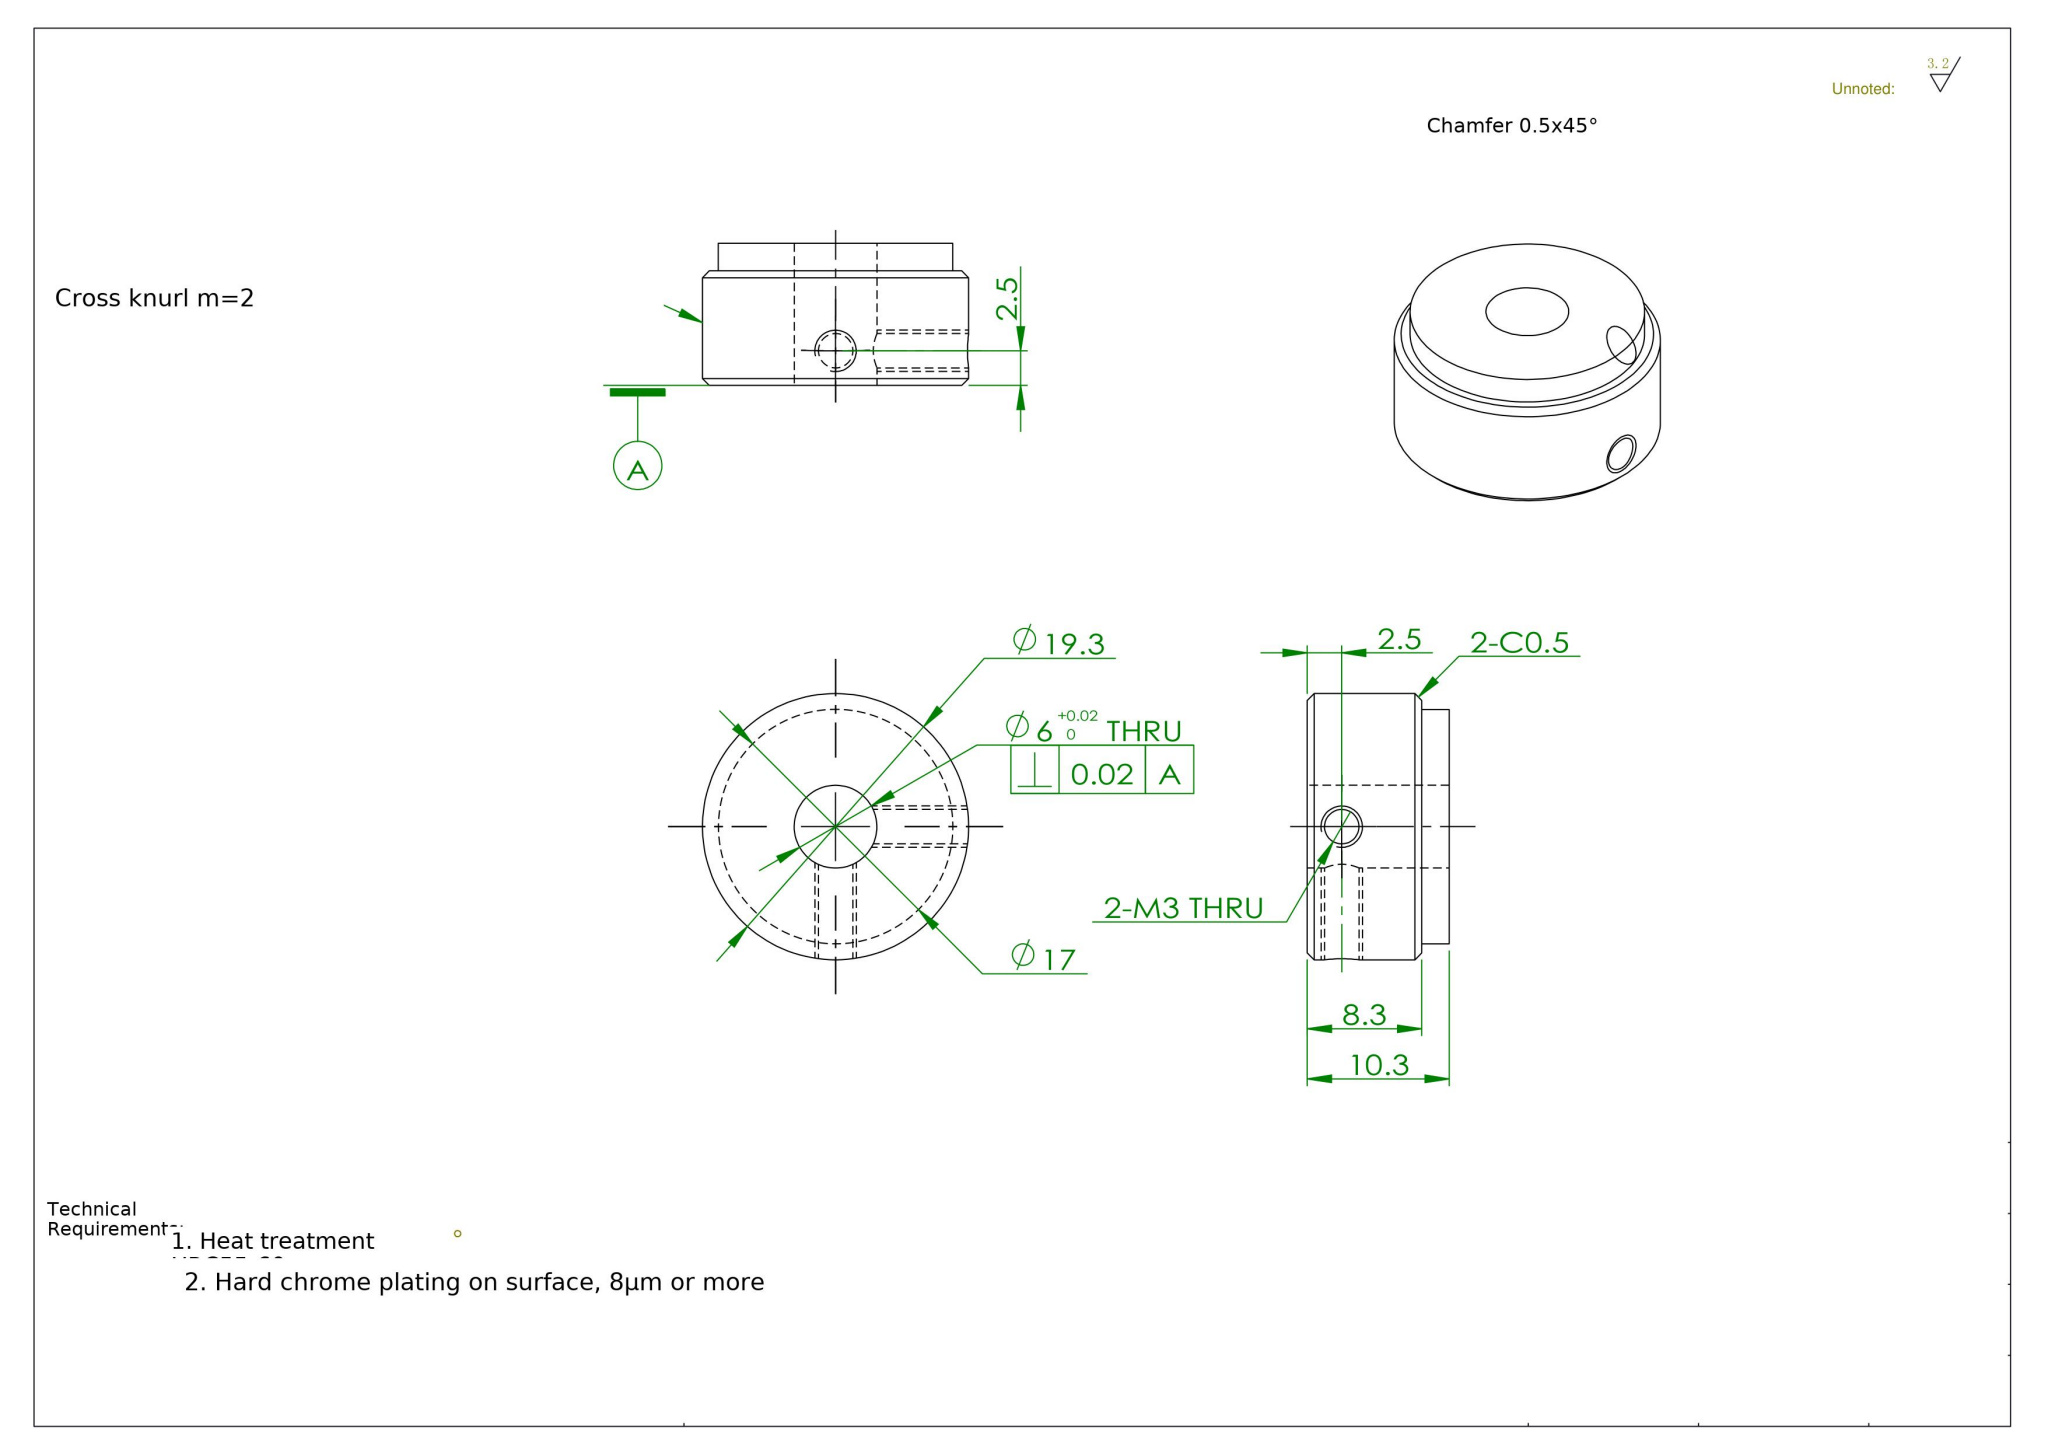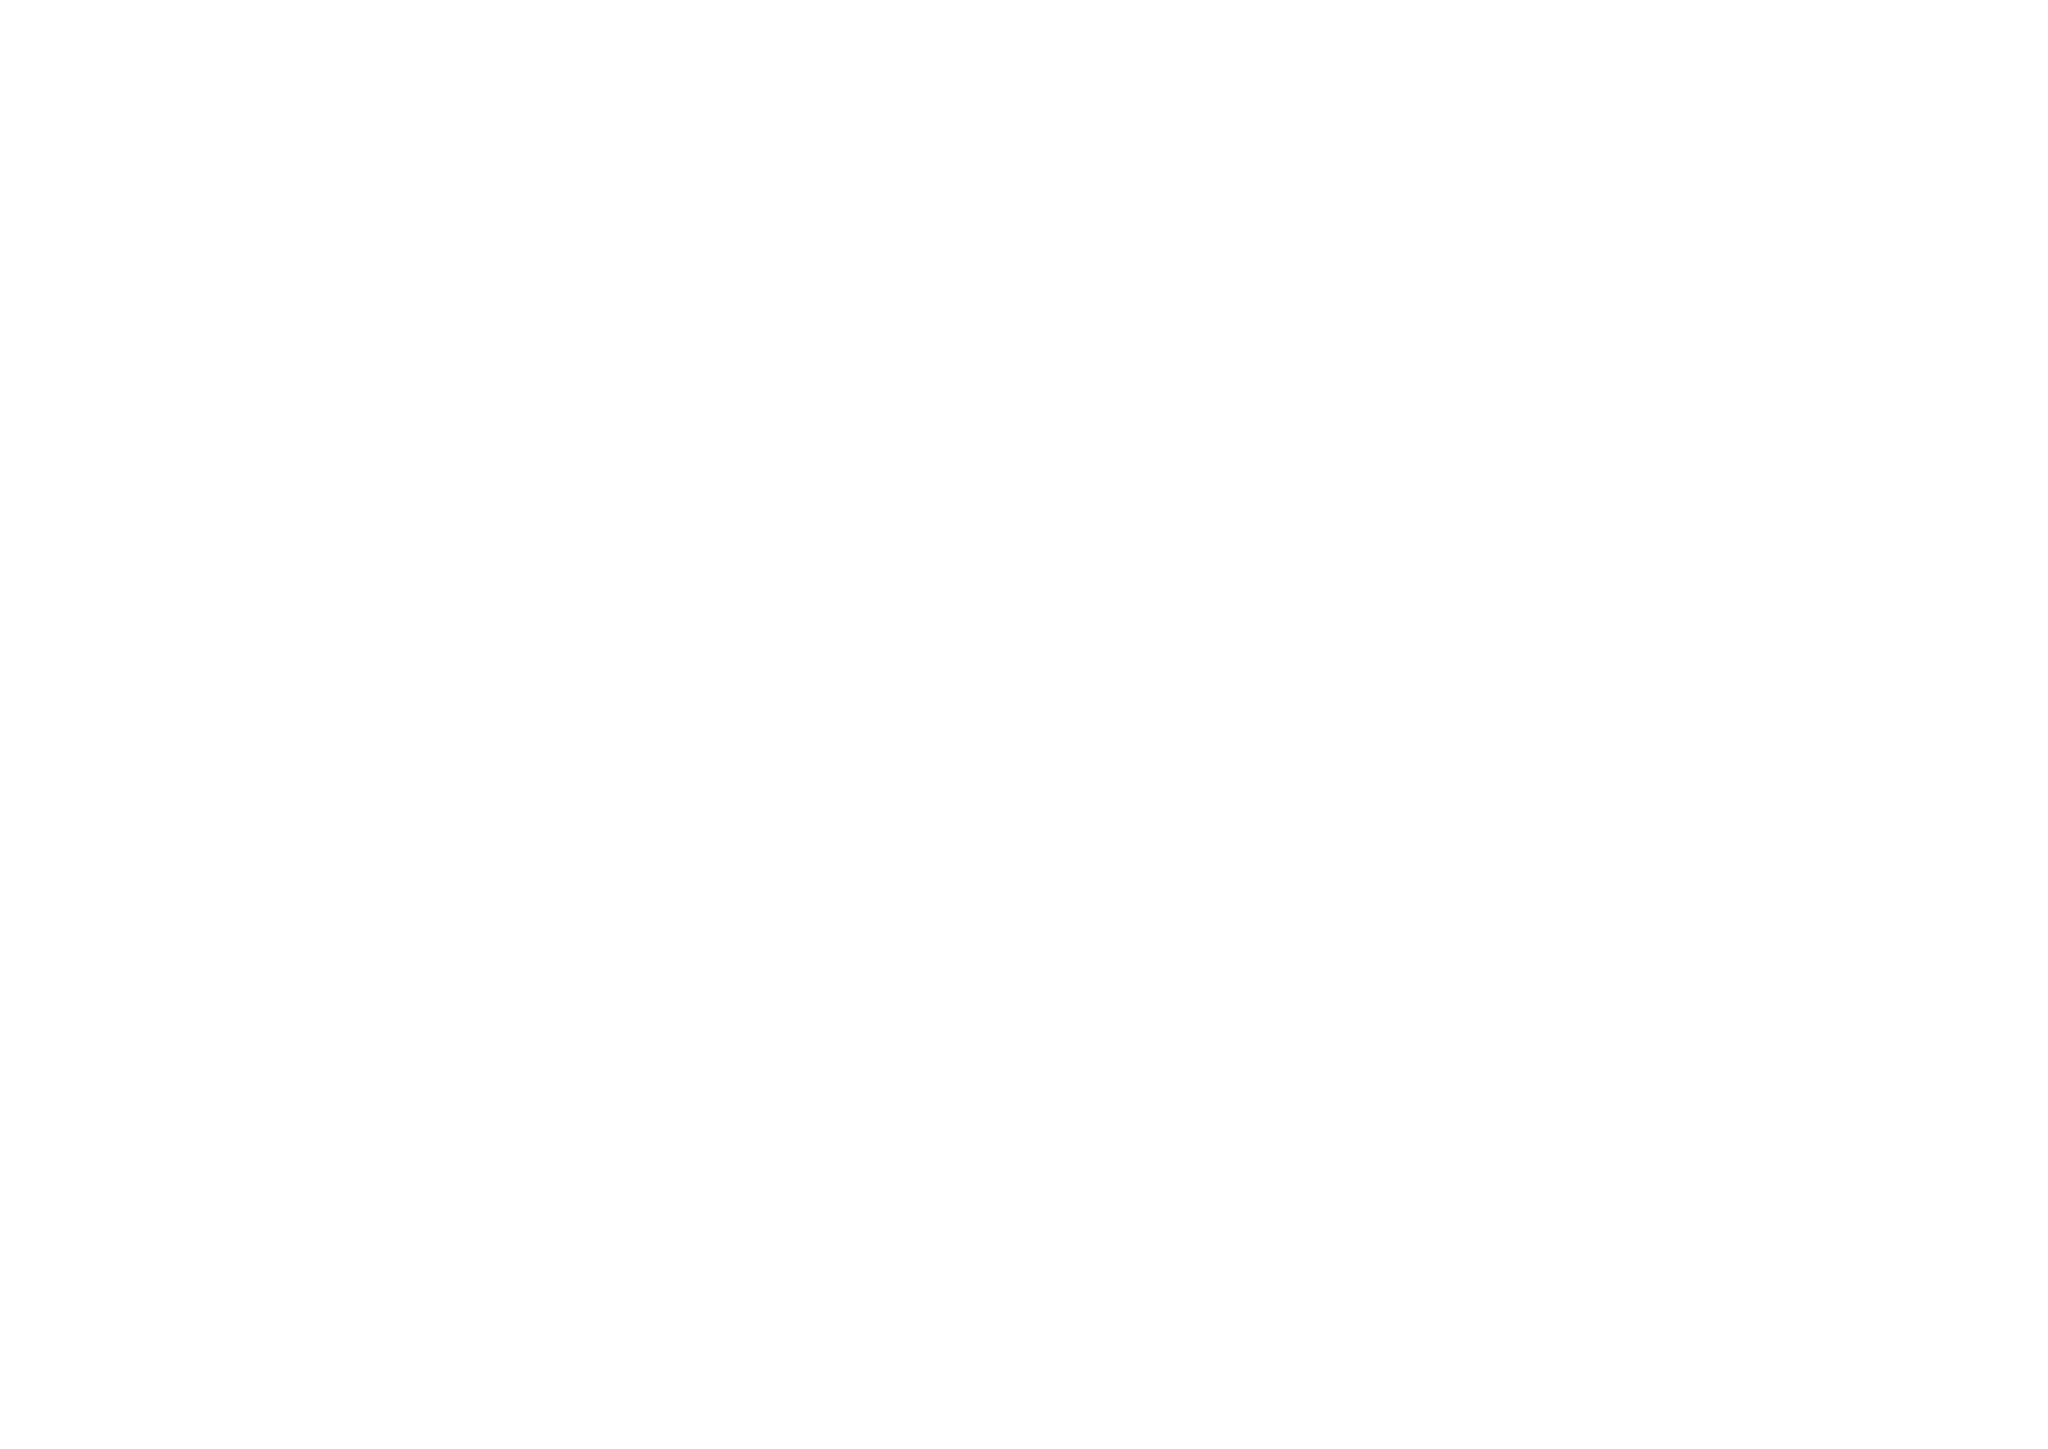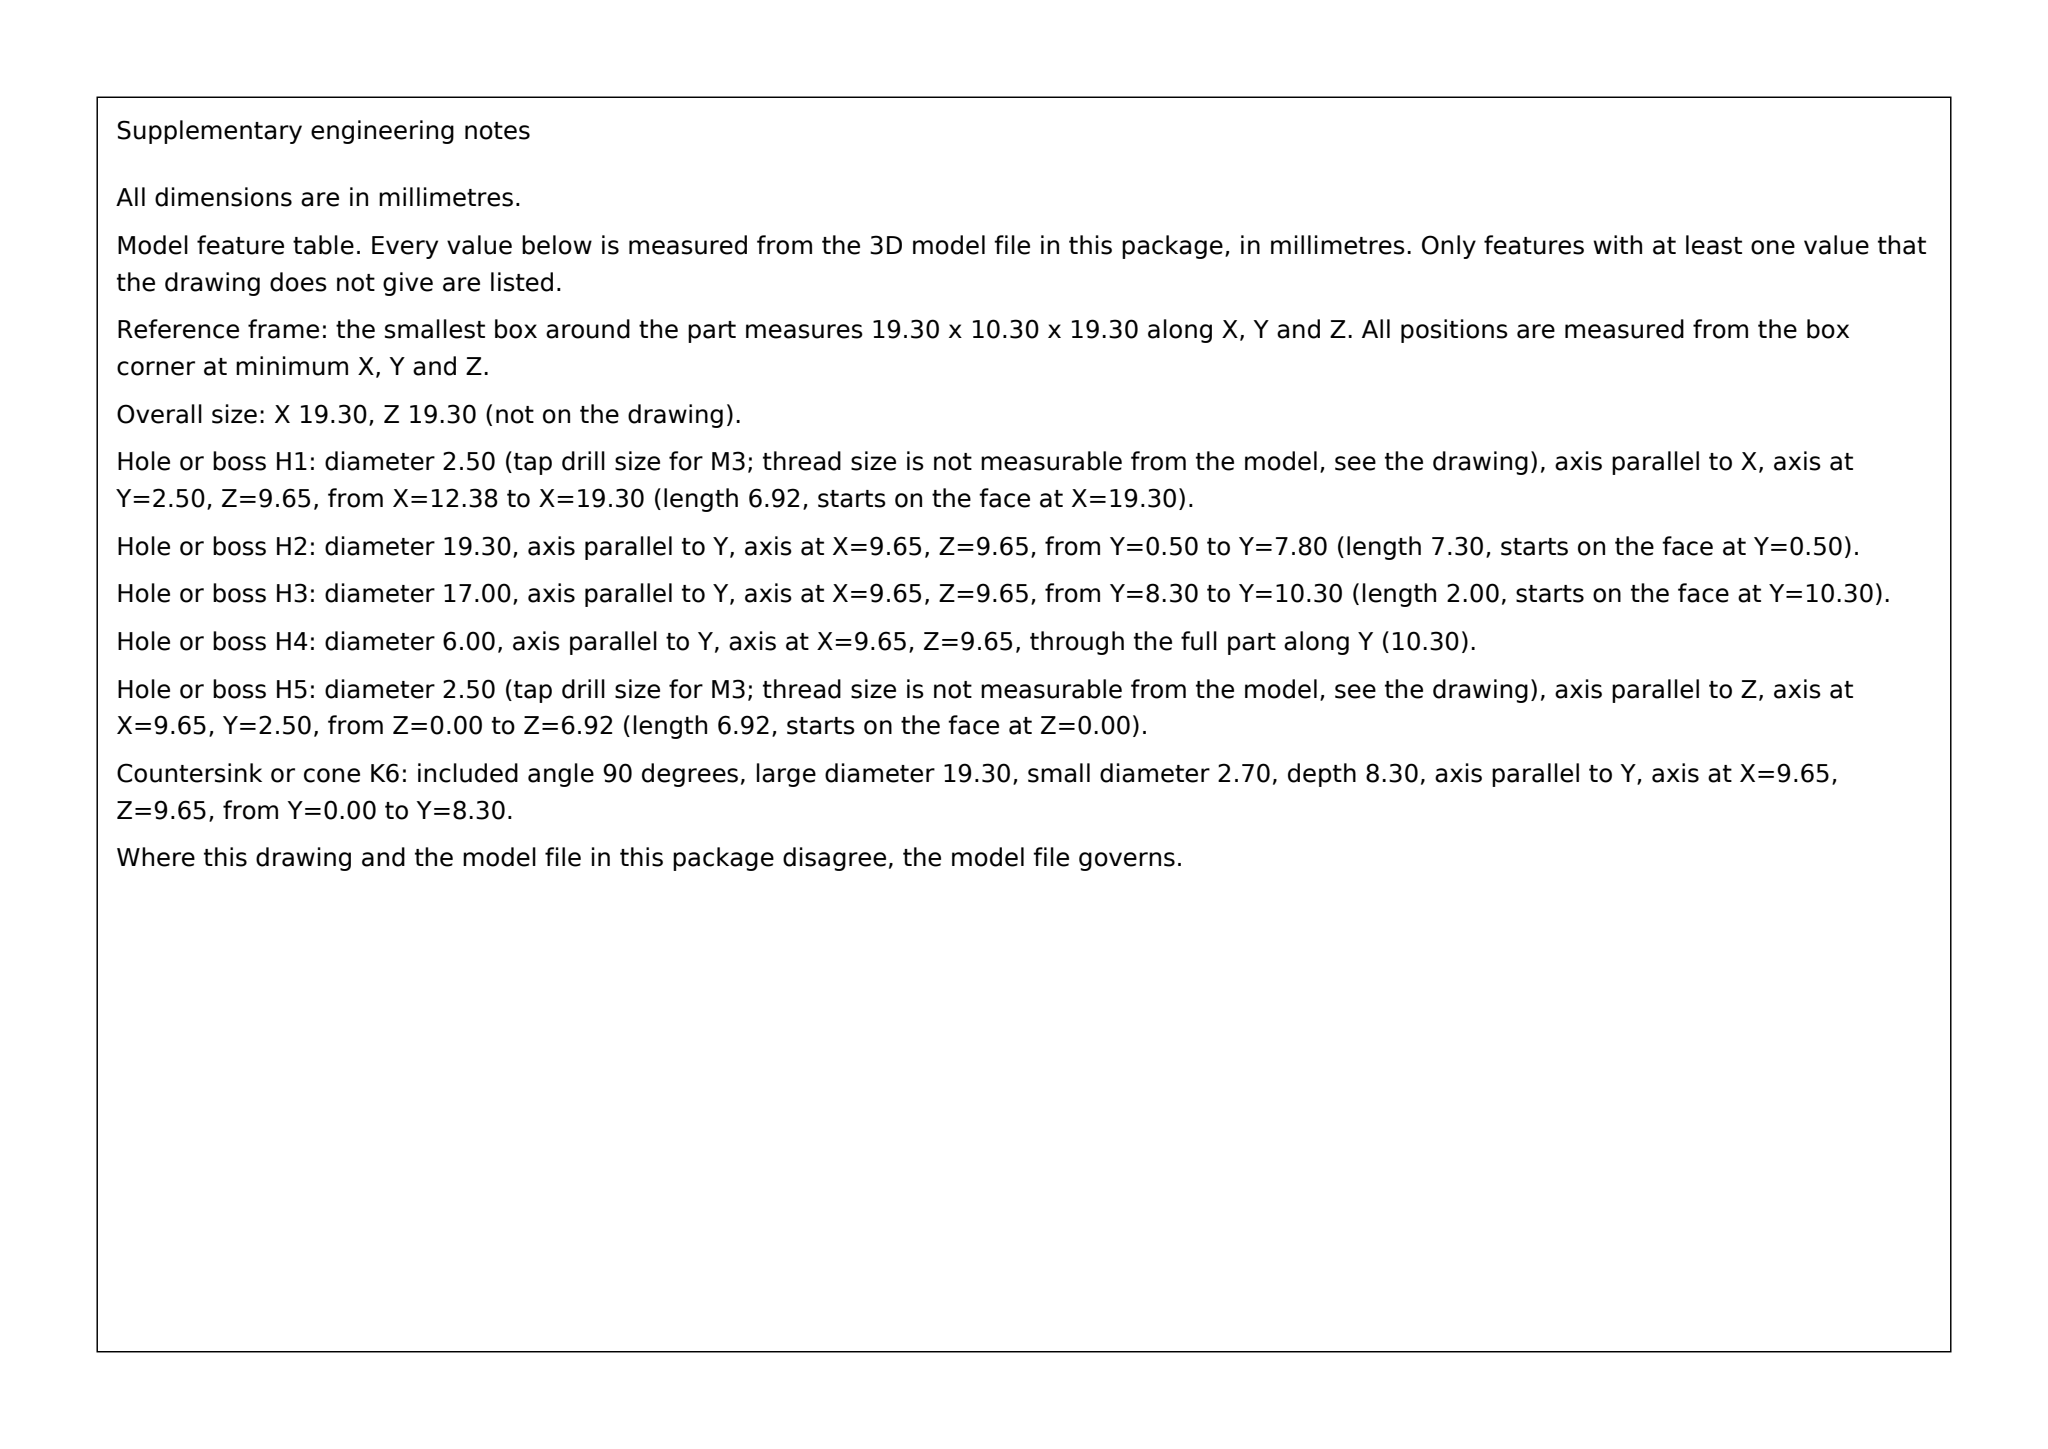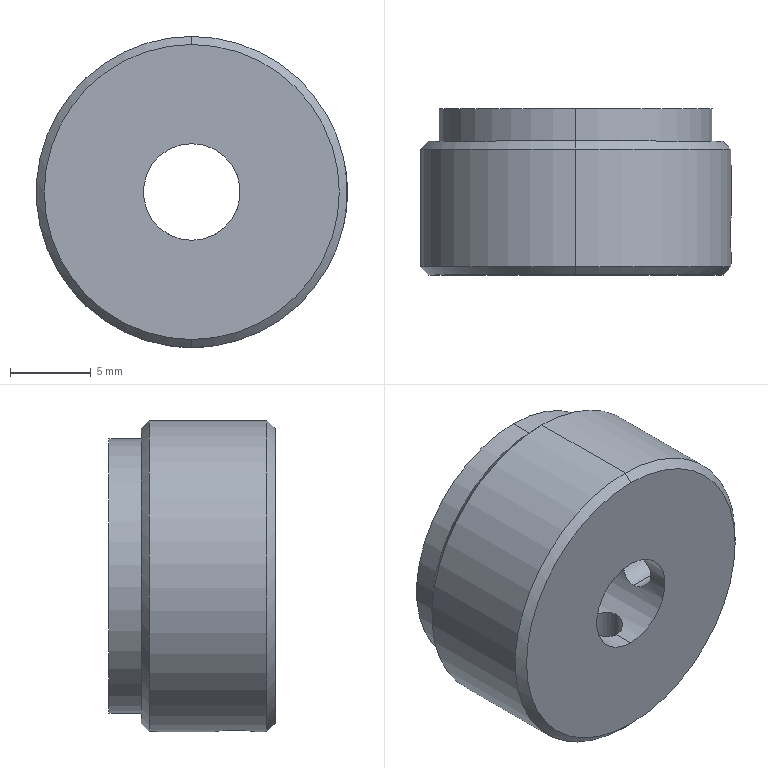Part | SolidWorks | mm | 1 solid | 17 faces | box 19.3 x 10.3 x 19.3 mm | volume 2510 mm3 | cylinder 10 | cone 4 | plane 3 | commonest cylinder face diameters 2.5 x4 19.3 x2 17 x2 6 x2
build123d program:
from build123d import *

# Parameters (mm, degrees)
M3_TAPPED_HOLE1_REACH  = 25.91
M3_TAPPED_HOLE1_BORE_R = 1.25
CIRPATTERN1_COUNT      = 2
CIRPATTERN1_ANGLE      = 90
CHAMFER1_SIZE          = 0.5


with BuildPart() as part:
    # Sketch1 → Revolve1 (revolve)
    with BuildSketch(Plane.XY, mode=Mode.PRIVATE) as revolve1_sk:
        Polygon((3, 0), (3, 10.3), (8.5, 10.3), (8.5, 8.3), (9.65, 8.3), (9.65, 0), align=None)
    revolve(revolve1_sk.sketch.rotate(Axis((0, 77.358, 0), (0, -1, 0)), 90), axis=Axis((0, 77.358, 0), (0, -1, 0)))

    # M3 Tapped Hole1 bore → M3 Tapped Hole1 (cut, up to next)
    with BuildSketch(Plane(origin=(9.65, 0, 0), x_dir=(0, 0, -1), z_dir=(1, 0, 0)), mode=Mode.PRIVATE) as m3_tapped_hole1_sk1:
        with Locations((0, 2.5)):
            Circle(M3_TAPPED_HOLE1_BORE_R)
    m3_tapped_hole1_tool1 = extrude(m3_tapped_hole1_sk1.sketch, amount=-M3_TAPPED_HOLE1_REACH, mode=Mode.PRIVATE) & part.part
    m3_tapped_hole1 = m3_tapped_hole1_tool1.solids().sort_by_distance((9.65, 2.5, 0))[0]
    add(m3_tapped_hole1, mode=Mode.SUBTRACT)

    # CirPattern1: M3 Tapped Hole1 ×2 about axis
    cirpattern1_axis = Axis((0, 77.358, 0), (0, 1, 0))
    for i in range(1, CIRPATTERN1_COUNT):
        add(m3_tapped_hole1.rotate(cirpattern1_axis, i * CIRPATTERN1_ANGLE / (CIRPATTERN1_COUNT - 1)), mode=Mode.SUBTRACT)

    # Chamfer1
    chamfer1_edges = [part.edges().sort_by_distance(p)[0] for p in [
        (0, 0, -9.65),
        (0, 8.3, -9.65),
    ]]
    chamfer(chamfer1_edges, length=CHAMFER1_SIZE)


solid = part.part